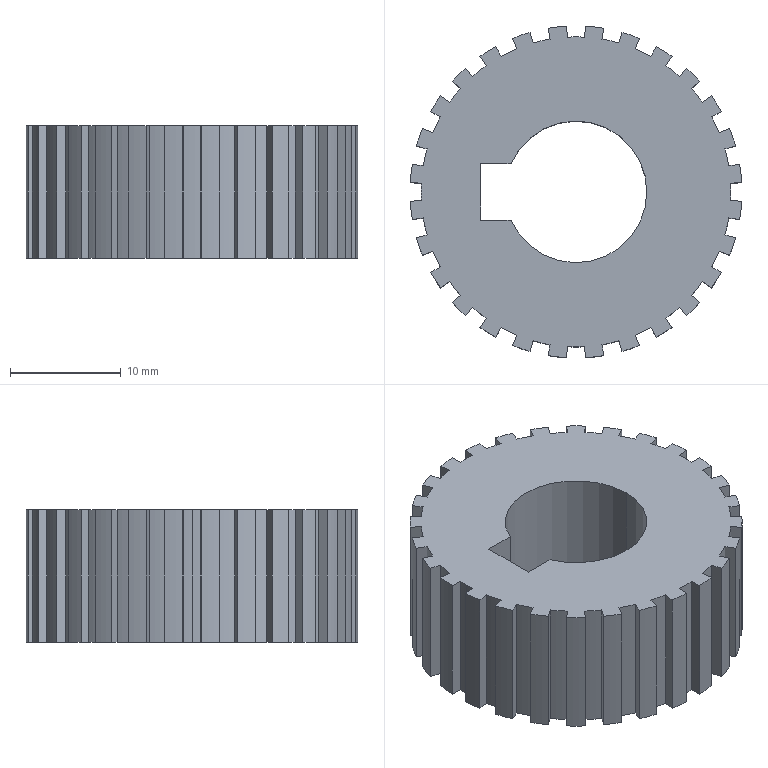Component | SolidWorks | Pulley11.1-1 | 1 solid | 120 faces | volume 6246 mm3 | plane 61 | cylinder 59 | commonest cylinder face diameters 28 x29 30 x28 12.8 x2